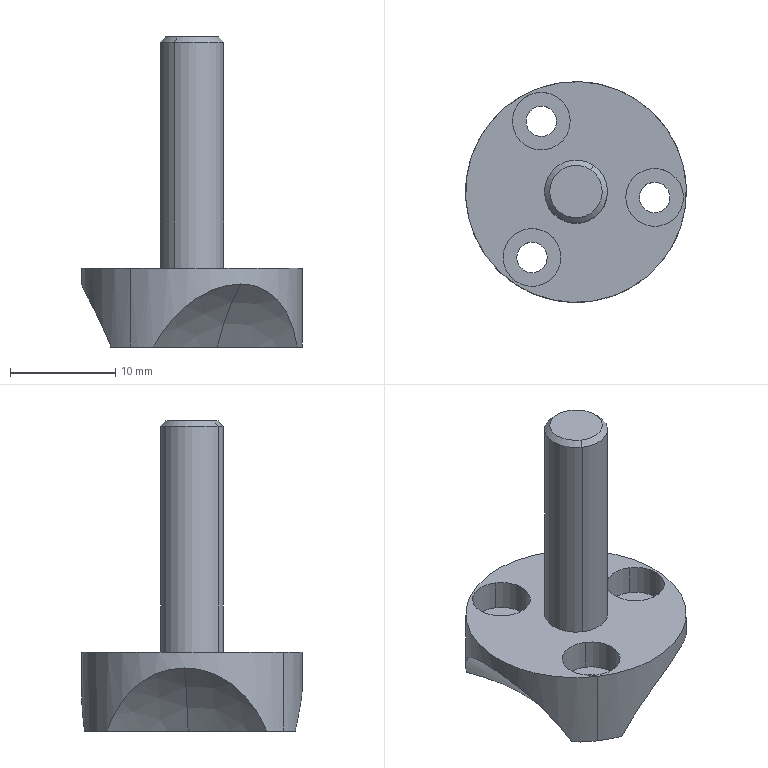Component | SolidWorks | Connector-1 | 1 solid | 33 faces | box 21 x 21 x 29.5 mm | volume 2358 mm3 | cylinder 18 | plane 7 | sphere 6 | cone 2 | commonest cylinder face diameters 5.5 x6 2.9 x6 10 x2 6 x2 21 x2
STEP:
#1=COLOUR_RGB('',0.7922,0.8196,0.9333);
#2=FILL_AREA_STYLE_COLOUR('',#1);
#3=FILL_AREA_STYLE('',(#2));
#4=SURFACE_STYLE_FILL_AREA(#3);
#5=SURFACE_SIDE_STYLE('',(#4));
#6=SURFACE_STYLE_USAGE(.BOTH.,#5);
#7=PRESENTATION_STYLE_ASSIGNMENT((#6));
#8=CARTESIAN_POINT('',(-8.497,3.918,42.455));
#9=VERTEX_POINT('',#8);
#10=CARTESIAN_POINT('',(-8.716,3.591,42.455));
#11=VERTEX_POINT('',#10);
#12=CARTESIAN_POINT('',(-8.607,3.755,42.455));
#13=DIRECTION('',(-0.,0.,-1.));
#14=DIRECTION('',(-0.5579,-0.8299,0.));
#15=AXIS2_PLACEMENT_3D('',#12,#13,#14);
#16=CIRCLE('',#15,0.1969);
#17=EDGE_CURVE('',#9,#11,#16,.T.);
#18=ORIENTED_EDGE('',*,*,#17,.F.);
#19=CARTESIAN_POINT('',(-8.497,3.918,42.396));
#20=VERTEX_POINT('',#19);
#21=CARTESIAN_POINT('',(-8.497,3.918,42.376));
#22=DIRECTION('',(-0.,0.,-1.));
#23=VECTOR('',#22,39.37);
#24=LINE('',#21,#23);
#25=EDGE_CURVE('',#9,#20,#24,.T.);
#26=ORIENTED_EDGE('',*,*,#25,.T.);
#27=CARTESIAN_POINT('',(-8.716,3.591,42.396));
#28=VERTEX_POINT('',#27);
#29=CARTESIAN_POINT('',(-8.607,3.755,42.396));
#30=DIRECTION('',(-0.,0.,-1.));
#31=DIRECTION('',(0.5579,0.8299,0.));
#32=AXIS2_PLACEMENT_3D('',#29,#30,#31);
#33=CIRCLE('',#32,0.1969);
#34=EDGE_CURVE('',#20,#28,#33,.T.);
#35=ORIENTED_EDGE('',*,*,#34,.T.);
#36=CARTESIAN_POINT('',(-8.716,3.591,42.376));
#37=DIRECTION('',(-0.,0.,-1.));
#38=VECTOR('',#37,39.37);
#39=LINE('',#36,#38);
#40=EDGE_CURVE('',#11,#28,#39,.T.);
#41=ORIENTED_EDGE('',*,*,#40,.F.);
#42=EDGE_LOOP('',(#18,#26,#35,#41));
#43=FACE_OUTER_BOUND('',#42,.T.);
#44=CARTESIAN_POINT('',(-8.607,3.755,42.376));
#45=DIRECTION('',(-0.,0.,-1.));
#46=DIRECTION('',(-0.5579,-0.8299,0.));
#47=AXIS2_PLACEMENT_3D('',#44,#45,#46);
#48=CYLINDRICAL_SURFACE('',#47,0.1969);
#49=ADVANCED_FACE('',(#43),#48,.F.);
#50=CARTESIAN_POINT('',(-8.821,3.769,42.396));
#51=VERTEX_POINT('',#50);
#52=CARTESIAN_POINT('',(-8.869,4.074,42.396));
#53=VERTEX_POINT('',#52);
#54=CARTESIAN_POINT('',(-9.51,3.816,42.396));
#55=DIRECTION('',(0.,-0.,1.));
#56=DIRECTION('',(0.5579,0.8299,0.));
#57=AXIS2_PLACEMENT_3D('',#54,#55,#56);
#58=CIRCLE('',#57,0.6906);
#59=EDGE_CURVE('',#51,#53,#58,.T.);
#60=ORIENTED_EDGE('',*,*,#59,.F.);
#61=CARTESIAN_POINT('',(-9.019,3.783,42.632));
#62=VERTEX_POINT('',#61);
#63=CARTESIAN_POINT('',(-9.51,3.816,42.017));
#64=DIRECTION('',(-0.06817,-0.9977,-0.));
#65=DIRECTION('',(0.9977,-0.06817,0.));
#66=AXIS2_PLACEMENT_3D('',#63,#64,#65);
#67=CIRCLE('',#66,0.7874);
#68=EDGE_CURVE('',#51,#62,#67,.T.);
#69=ORIENTED_EDGE('',*,*,#68,.T.);
#70=CARTESIAN_POINT('',(-9.019,3.783,42.632));
#71=CARTESIAN_POINT('',(-9.018,3.792,42.632));
#72=CARTESIAN_POINT('',(-9.017,3.801,42.631));
#73=CARTESIAN_POINT('',(-9.015,3.819,42.63));
#74=CARTESIAN_POINT('',(-9.014,3.827,42.628));
#75=CARTESIAN_POINT('',(-9.01,3.845,42.625));
#76=CARTESIAN_POINT('',(-9.008,3.853,42.623));
#77=CARTESIAN_POINT('',(-9.004,3.87,42.618));
#78=CARTESIAN_POINT('',(-9.001,3.878,42.615));
#79=CARTESIAN_POINT('',(-8.993,3.902,42.605));
#80=CARTESIAN_POINT('',(-8.987,3.917,42.598));
#81=CARTESIAN_POINT('',(-8.977,3.938,42.584));
#82=CARTESIAN_POINT('',(-8.974,3.945,42.579));
#83=CARTESIAN_POINT('',(-8.967,3.958,42.569));
#84=CARTESIAN_POINT('',(-8.963,3.964,42.564));
#85=CARTESIAN_POINT('',(-8.952,3.982,42.548));
#86=CARTESIAN_POINT('',(-8.944,3.993,42.536));
#87=CARTESIAN_POINT('',(-8.929,4.014,42.511));
#88=CARTESIAN_POINT('',(-8.921,4.023,42.498));
#89=CARTESIAN_POINT('',(-8.898,4.049,42.456));
#90=CARTESIAN_POINT('',(-8.883,4.062,42.427));
#91=CARTESIAN_POINT('',(-8.869,4.074,42.396));
#92=B_SPLINE_CURVE_WITH_KNOTS('',3,(#70,#71,#72,#73,#74,#75,#76,#77,#78,#79,#80,#81,#82,#83,#84,#85,#86,#87,#88,#89,#90,#91),.UNSPECIFIED.,.F.,.F.,(4,2,2,2,2,2,2,2,2,2,4),(0.01143,0.0121,0.01278,0.01346,0.01414,0.01549,0.01617,0.01684,0.0182,0.01955,0.02226),.UNSPECIFIED.);
#93=EDGE_CURVE('',#62,#53,#92,.T.);
#94=ORIENTED_EDGE('',*,*,#93,.T.);
#95=EDGE_LOOP('',(#60,#69,#94));
#96=FACE_OUTER_BOUND('',#95,.T.);
#97=CARTESIAN_POINT('',(-9.51,3.816,42.017));
#98=DIRECTION('',(0.06817,0.9977,0.));
#99=DIRECTION('',(0.9977,-0.06817,0.));
#100=AXIS2_PLACEMENT_3D('',#97,#98,#99);
#101=SPHERICAL_SURFACE('',#100,0.7874);
#102=ADVANCED_FACE('',(#96),#101,.F.);
#103=CARTESIAN_POINT('',(-8.512,3.561,42.396));
#104=VERTEX_POINT('',#103);
#105=CARTESIAN_POINT('',(-8.751,3.367,42.396));
#106=VERTEX_POINT('',#105);
#107=CARTESIAN_POINT('',(-8.208,2.941,42.396));
#108=DIRECTION('',(0.,-0.,1.));
#109=DIRECTION('',(0.5579,0.8299,0.));
#110=AXIS2_PLACEMENT_3D('',#107,#108,#109);
#111=CIRCLE('',#110,0.6906);
#112=EDGE_CURVE('',#104,#106,#111,.T.);
#113=ORIENTED_EDGE('',*,*,#112,.F.);
#114=CARTESIAN_POINT('',(-8.425,3.383,42.632));
#115=VERTEX_POINT('',#114);
#116=CARTESIAN_POINT('',(-8.208,2.941,42.017));
#117=DIRECTION('',(0.8981,0.4398,-0.));
#118=DIRECTION('',(-0.4398,0.8981,0.));
#119=AXIS2_PLACEMENT_3D('',#116,#117,#118);
#120=CIRCLE('',#119,0.7874);
#121=EDGE_CURVE('',#104,#115,#120,.T.);
#122=ORIENTED_EDGE('',*,*,#121,.T.);
#123=CARTESIAN_POINT('',(-8.425,3.383,42.632));
#124=CARTESIAN_POINT('',(-8.433,3.379,42.632));
#125=CARTESIAN_POINT('',(-8.441,3.376,42.631));
#126=CARTESIAN_POINT('',(-8.458,3.369,42.63));
#127=CARTESIAN_POINT('',(-8.466,3.366,42.628));
#128=CARTESIAN_POINT('',(-8.483,3.36,42.625));
#129=CARTESIAN_POINT('',(-8.491,3.358,42.623));
#130=CARTESIAN_POINT('',(-8.508,3.353,42.618));
#131=CARTESIAN_POINT('',(-8.516,3.351,42.615));
#132=CARTESIAN_POINT('',(-8.541,3.346,42.605));
#133=CARTESIAN_POINT('',(-8.557,3.344,42.598));
#134=CARTESIAN_POINT('',(-8.58,3.342,42.584));
#135=CARTESIAN_POINT('',(-8.588,3.342,42.579));
#136=CARTESIAN_POINT('',(-8.603,3.341,42.569));
#137=CARTESIAN_POINT('',(-8.61,3.341,42.564));
#138=CARTESIAN_POINT('',(-8.631,3.342,42.548));
#139=CARTESIAN_POINT('',(-8.644,3.343,42.536));
#140=CARTESIAN_POINT('',(-8.67,3.346,42.511));
#141=CARTESIAN_POINT('',(-8.682,3.348,42.498));
#142=CARTESIAN_POINT('',(-8.715,3.355,42.456));
#143=CARTESIAN_POINT('',(-8.735,3.361,42.427));
#144=CARTESIAN_POINT('',(-8.751,3.367,42.396));
#145=B_SPLINE_CURVE_WITH_KNOTS('',3,(#123,#124,#125,#126,#127,#128,#129,#130,#131,#132,#133,#134,#135,#136,#137,#138,#139,#140,#141,#142,#143,#144),.UNSPECIFIED.,.F.,.F.,(4,2,2,2,2,2,2,2,2,2,4),(0.01143,0.0121,0.01278,0.01346,0.01414,0.01549,0.01617,0.01684,0.0182,0.01955,0.02226),.UNSPECIFIED.);
#146=EDGE_CURVE('',#115,#106,#145,.T.);
#147=ORIENTED_EDGE('',*,*,#146,.T.);
#148=EDGE_LOOP('',(#113,#122,#147));
#149=FACE_OUTER_BOUND('',#148,.T.);
#150=CARTESIAN_POINT('',(-8.208,2.941,42.017));
#151=DIRECTION('',(-0.8981,-0.4398,0.));
#152=DIRECTION('',(-0.4398,0.8981,0.));
#153=AXIS2_PLACEMENT_3D('',#150,#151,#152);
#154=SPHERICAL_SURFACE('',#153,0.7874);
#155=ADVANCED_FACE('',(#149),#154,.F.);
#156=CARTESIAN_POINT('',(-8.487,3.933,42.396));
#157=VERTEX_POINT('',#156);
#158=CARTESIAN_POINT('',(-8.199,3.823,42.396));
#159=VERTEX_POINT('',#158);
#160=CARTESIAN_POINT('',(-8.101,4.506,42.396));
#161=DIRECTION('',(0.,-0.,1.));
#162=DIRECTION('',(0.5579,0.8299,0.));
#163=AXIS2_PLACEMENT_3D('',#160,#161,#162);
#164=CIRCLE('',#163,0.6906);
#165=EDGE_CURVE('',#157,#159,#164,.T.);
#166=ORIENTED_EDGE('',*,*,#165,.F.);
#167=CARTESIAN_POINT('',(-8.376,4.098,42.632));
#168=VERTEX_POINT('',#167);
#169=CARTESIAN_POINT('',(-8.101,4.506,42.017));
#170=DIRECTION('',(-0.8299,0.5579,0.));
#171=DIRECTION('',(-0.5579,-0.8299,0.));
#172=AXIS2_PLACEMENT_3D('',#169,#170,#171);
#173=CIRCLE('',#172,0.7874);
#174=EDGE_CURVE('',#157,#168,#173,.T.);
#175=ORIENTED_EDGE('',*,*,#174,.T.);
#176=CARTESIAN_POINT('',(-8.376,4.098,42.632));
#177=CARTESIAN_POINT('',(-8.368,4.093,42.632));
#178=CARTESIAN_POINT('',(-8.361,4.087,42.631));
#179=CARTESIAN_POINT('',(-8.347,4.076,42.63));
#180=CARTESIAN_POINT('',(-8.34,4.071,42.628));
#181=CARTESIAN_POINT('',(-8.327,4.059,42.625));
#182=CARTESIAN_POINT('',(-8.321,4.053,42.623));
#183=CARTESIAN_POINT('',(-8.308,4.041,42.618));
#184=CARTESIAN_POINT('',(-8.302,4.035,42.615));
#185=CARTESIAN_POINT('',(-8.286,4.016,42.605));
#186=CARTESIAN_POINT('',(-8.276,4.003,42.598));
#187=CARTESIAN_POINT('',(-8.262,3.984,42.584));
#188=CARTESIAN_POINT('',(-8.258,3.977,42.579));
#189=CARTESIAN_POINT('',(-8.25,3.965,42.569));
#190=CARTESIAN_POINT('',(-8.247,3.958,42.564));
#191=CARTESIAN_POINT('',(-8.237,3.94,42.548));
#192=CARTESIAN_POINT('',(-8.231,3.928,42.536));
#193=CARTESIAN_POINT('',(-8.221,3.904,42.511));
#194=CARTESIAN_POINT('',(-8.217,3.893,42.498));
#195=CARTESIAN_POINT('',(-8.206,3.86,42.456));
#196=CARTESIAN_POINT('',(-8.202,3.84,42.427));
#197=CARTESIAN_POINT('',(-8.199,3.823,42.396));
#198=B_SPLINE_CURVE_WITH_KNOTS('',3,(#176,#177,#178,#179,#180,#181,#182,#183,#184,#185,#186,#187,#188,#189,#190,#191,#192,#193,#194,#195,#196,#197),.UNSPECIFIED.,.F.,.F.,(4,2,2,2,2,2,2,2,2,2,4),(0.01143,0.0121,0.01278,0.01346,0.01414,0.01549,0.01617,0.01684,0.0182,0.01955,0.02226),.UNSPECIFIED.);
#199=EDGE_CURVE('',#168,#159,#198,.T.);
#200=ORIENTED_EDGE('',*,*,#199,.T.);
#201=EDGE_LOOP('',(#166,#175,#200));
#202=FACE_OUTER_BOUND('',#201,.T.);
#203=CARTESIAN_POINT('',(-8.101,4.506,42.017));
#204=DIRECTION('',(0.8299,-0.5579,-0.));
#205=DIRECTION('',(-0.5579,-0.8299,0.));
#206=AXIS2_PLACEMENT_3D('',#203,#204,#205);
#207=SPHERICAL_SURFACE('',#206,0.7874);
#208=ADVANCED_FACE('',(#202),#207,.F.);
#209=CARTESIAN_POINT('',(-8.832,3.42,42.577));
#210=VERTEX_POINT('',#209);
#211=CARTESIAN_POINT('',(-8.711,3.599,42.577));
#212=VERTEX_POINT('',#211);
#213=CARTESIAN_POINT('',(-8.771,3.51,42.577));
#214=DIRECTION('',(0.,-0.,1.));
#215=DIRECTION('',(0.5579,0.8299,0.));
#216=AXIS2_PLACEMENT_3D('',#213,#214,#215);
#217=CIRCLE('',#216,0.1083);
#218=EDGE_CURVE('',#210,#212,#217,.T.);
#219=ORIENTED_EDGE('',*,*,#218,.F.);
#220=CARTESIAN_POINT('',(-8.832,3.42,42.691));
#221=VERTEX_POINT('',#220);
#222=CARTESIAN_POINT('',(-8.832,3.42,42.691));
#223=DIRECTION('',(0.,-0.,1.));
#224=VECTOR('',#223,39.37);
#225=LINE('',#222,#224);
#226=EDGE_CURVE('',#210,#221,#225,.T.);
#227=ORIENTED_EDGE('',*,*,#226,.T.);
#228=CARTESIAN_POINT('',(-8.711,3.599,42.691));
#229=VERTEX_POINT('',#228);
#230=CARTESIAN_POINT('',(-8.771,3.51,42.691));
#231=DIRECTION('',(0.,-0.,1.));
#232=DIRECTION('',(0.5579,0.8299,0.));
#233=AXIS2_PLACEMENT_3D('',#230,#231,#232);
#234=CIRCLE('',#233,0.1083);
#235=EDGE_CURVE('',#221,#229,#234,.T.);
#236=ORIENTED_EDGE('',*,*,#235,.T.);
#237=CARTESIAN_POINT('',(-8.711,3.599,42.691));
#238=DIRECTION('',(0.,-0.,1.));
#239=VECTOR('',#238,39.37);
#240=LINE('',#237,#239);
#241=EDGE_CURVE('',#212,#229,#240,.T.);
#242=ORIENTED_EDGE('',*,*,#241,.F.);
#243=EDGE_LOOP('',(#219,#227,#236,#242));
#244=FACE_OUTER_BOUND('',#243,.T.);
#245=CARTESIAN_POINT('',(-8.771,3.51,42.691));
#246=DIRECTION('',(0.,-0.,1.));
#247=DIRECTION('',(0.5579,0.8299,0.));
#248=AXIS2_PLACEMENT_3D('',#245,#246,#247);
#249=CYLINDRICAL_SURFACE('',#248,0.1083);
#250=ADVANCED_FACE('',(#244),#249,.F.);
#251=CARTESIAN_POINT('',(-8.739,3.557,42.396));
#252=VERTEX_POINT('',#251);
#253=CARTESIAN_POINT('',(-8.803,3.462,42.396));
#254=VERTEX_POINT('',#253);
#255=CARTESIAN_POINT('',(-8.771,3.51,42.396));
#256=DIRECTION('',(-0.,0.,-1.));
#257=DIRECTION('',(0.5579,0.8299,0.));
#258=AXIS2_PLACEMENT_3D('',#255,#256,#257);
#259=CIRCLE('',#258,0.05709);
#260=EDGE_CURVE('',#252,#254,#259,.T.);
#261=ORIENTED_EDGE('',*,*,#260,.T.);
#262=CARTESIAN_POINT('',(-8.803,3.462,42.577));
#263=VERTEX_POINT('',#262);
#264=CARTESIAN_POINT('',(-8.803,3.462,42.691));
#265=DIRECTION('',(0.,-0.,1.));
#266=VECTOR('',#265,39.37);
#267=LINE('',#264,#266);
#268=EDGE_CURVE('',#254,#263,#267,.T.);
#269=ORIENTED_EDGE('',*,*,#268,.T.);
#270=CARTESIAN_POINT('',(-8.739,3.557,42.577));
#271=VERTEX_POINT('',#270);
#272=CARTESIAN_POINT('',(-8.771,3.51,42.577));
#273=DIRECTION('',(0.,-0.,1.));
#274=DIRECTION('',(0.5579,0.8299,0.));
#275=AXIS2_PLACEMENT_3D('',#272,#273,#274);
#276=CIRCLE('',#275,0.05709);
#277=EDGE_CURVE('',#263,#271,#276,.T.);
#278=ORIENTED_EDGE('',*,*,#277,.T.);
#279=CARTESIAN_POINT('',(-8.739,3.557,42.691));
#280=DIRECTION('',(0.,-0.,1.));
#281=VECTOR('',#280,39.37);
#282=LINE('',#279,#281);
#283=EDGE_CURVE('',#252,#271,#282,.T.);
#284=ORIENTED_EDGE('',*,*,#283,.F.);
#285=EDGE_LOOP('',(#261,#269,#278,#284));
#286=FACE_OUTER_BOUND('',#285,.T.);
#287=CARTESIAN_POINT('',(-8.771,3.51,42.691));
#288=DIRECTION('',(0.,-0.,1.));
#289=DIRECTION('',(0.5579,0.8299,0.));
#290=AXIS2_PLACEMENT_3D('',#287,#288,#289);
#291=CYLINDRICAL_SURFACE('',#290,0.05709);
#292=ADVANCED_FACE('',(#286),#291,.F.);
#293=CARTESIAN_POINT('',(-8.797,3.93,42.577));
#294=VERTEX_POINT('',#293);
#295=CARTESIAN_POINT('',(-8.676,4.11,42.577));
#296=VERTEX_POINT('',#295);
#297=CARTESIAN_POINT('',(-8.736,4.02,42.577));
#298=DIRECTION('',(0.,-0.,1.));
#299=DIRECTION('',(0.5579,0.8299,0.));
#300=AXIS2_PLACEMENT_3D('',#297,#298,#299);
#301=CIRCLE('',#300,0.1083);
#302=EDGE_CURVE('',#294,#296,#301,.T.);
#303=ORIENTED_EDGE('',*,*,#302,.F.);
#304=CARTESIAN_POINT('',(-8.797,3.93,42.691));
#305=VERTEX_POINT('',#304);
#306=CARTESIAN_POINT('',(-8.797,3.93,42.691));
#307=DIRECTION('',(0.,-0.,1.));
#308=VECTOR('',#307,39.37);
#309=LINE('',#306,#308);
#310=EDGE_CURVE('',#294,#305,#309,.T.);
#311=ORIENTED_EDGE('',*,*,#310,.T.);
#312=CARTESIAN_POINT('',(-8.676,4.11,42.691));
#313=VERTEX_POINT('',#312);
#314=CARTESIAN_POINT('',(-8.736,4.02,42.691));
#315=DIRECTION('',(0.,-0.,1.));
#316=DIRECTION('',(0.5579,0.8299,0.));
#317=AXIS2_PLACEMENT_3D('',#314,#315,#316);
#318=CIRCLE('',#317,0.1083);
#319=EDGE_CURVE('',#305,#313,#318,.T.);
#320=ORIENTED_EDGE('',*,*,#319,.T.);
#321=CARTESIAN_POINT('',(-8.676,4.11,42.691));
#322=DIRECTION('',(0.,-0.,1.));
#323=VECTOR('',#322,39.37);
#324=LINE('',#321,#323);
#325=EDGE_CURVE('',#296,#313,#324,.T.);
#326=ORIENTED_EDGE('',*,*,#325,.F.);
#327=EDGE_LOOP('',(#303,#311,#320,#326));
#328=FACE_OUTER_BOUND('',#327,.T.);
#329=CARTESIAN_POINT('',(-8.736,4.02,42.691));
#330=DIRECTION('',(0.,-0.,1.));
#331=DIRECTION('',(0.5579,0.8299,0.));
#332=AXIS2_PLACEMENT_3D('',#329,#330,#331);
#333=CYLINDRICAL_SURFACE('',#332,0.1083);
#334=ADVANCED_FACE('',(#328),#333,.F.);
#335=CARTESIAN_POINT('',(-8.705,4.067,42.396));
#336=VERTEX_POINT('',#335);
#337=CARTESIAN_POINT('',(-8.768,3.972,42.396));
#338=VERTEX_POINT('',#337);
#339=CARTESIAN_POINT('',(-8.736,4.02,42.396));
#340=DIRECTION('',(-0.,0.,-1.));
#341=DIRECTION('',(0.5579,0.8299,0.));
#342=AXIS2_PLACEMENT_3D('',#339,#340,#341);
#343=CIRCLE('',#342,0.05709);
#344=EDGE_CURVE('',#336,#338,#343,.T.);
#345=ORIENTED_EDGE('',*,*,#344,.T.);
#346=CARTESIAN_POINT('',(-8.768,3.972,42.577));
#347=VERTEX_POINT('',#346);
#348=CARTESIAN_POINT('',(-8.768,3.972,42.691));
#349=DIRECTION('',(0.,-0.,1.));
#350=VECTOR('',#349,39.37);
#351=LINE('',#348,#350);
#352=EDGE_CURVE('',#338,#347,#351,.T.);
#353=ORIENTED_EDGE('',*,*,#352,.T.);
#354=CARTESIAN_POINT('',(-8.705,4.067,42.577));
#355=VERTEX_POINT('',#354);
#356=CARTESIAN_POINT('',(-8.736,4.02,42.577));
#357=DIRECTION('',(0.,-0.,1.));
#358=DIRECTION('',(0.5579,0.8299,0.));
#359=AXIS2_PLACEMENT_3D('',#356,#357,#358);
#360=CIRCLE('',#359,0.05709);
#361=EDGE_CURVE('',#347,#355,#360,.T.);
#362=ORIENTED_EDGE('',*,*,#361,.T.);
#363=CARTESIAN_POINT('',(-8.705,4.067,42.691));
#364=DIRECTION('',(0.,-0.,1.));
#365=VECTOR('',#364,39.37);
#366=LINE('',#363,#365);
#367=EDGE_CURVE('',#336,#355,#366,.T.);
#368=ORIENTED_EDGE('',*,*,#367,.F.);
#369=EDGE_LOOP('',(#345,#353,#362,#368));
#370=FACE_OUTER_BOUND('',#369,.T.);
#371=CARTESIAN_POINT('',(-8.736,4.02,42.691));
#372=DIRECTION('',(0.,-0.,1.));
#373=DIRECTION('',(0.5579,0.8299,0.));
#374=AXIS2_PLACEMENT_3D('',#371,#372,#373);
#375=CYLINDRICAL_SURFACE('',#374,0.05709);
#376=ADVANCED_FACE('',(#370),#375,.F.);
#377=CARTESIAN_POINT('',(-8.372,3.645,42.577));
#378=VERTEX_POINT('',#377);
#379=CARTESIAN_POINT('',(-8.252,3.824,42.577));
#380=VERTEX_POINT('',#379);
#381=CARTESIAN_POINT('',(-8.312,3.734,42.577));
#382=DIRECTION('',(0.,-0.,1.));
#383=DIRECTION('',(0.5579,0.8299,0.));
#384=AXIS2_PLACEMENT_3D('',#381,#382,#383);
#385=CIRCLE('',#384,0.1083);
#386=EDGE_CURVE('',#378,#380,#385,.T.);
#387=ORIENTED_EDGE('',*,*,#386,.F.);
#388=CARTESIAN_POINT('',(-8.372,3.645,42.691));
#389=VERTEX_POINT('',#388);
#390=CARTESIAN_POINT('',(-8.372,3.645,42.691));
#391=DIRECTION('',(0.,-0.,1.));
#392=VECTOR('',#391,39.37);
#393=LINE('',#390,#392);
#394=EDGE_CURVE('',#378,#389,#393,.T.);
#395=ORIENTED_EDGE('',*,*,#394,.T.);
#396=CARTESIAN_POINT('',(-8.252,3.824,42.691));
#397=VERTEX_POINT('',#396);
#398=CARTESIAN_POINT('',(-8.312,3.734,42.691));
#399=DIRECTION('',(0.,-0.,1.));
#400=DIRECTION('',(0.5579,0.8299,0.));
#401=AXIS2_PLACEMENT_3D('',#398,#399,#400);
#402=CIRCLE('',#401,0.1083);
#403=EDGE_CURVE('',#389,#397,#402,.T.);
#404=ORIENTED_EDGE('',*,*,#403,.T.);
#405=CARTESIAN_POINT('',(-8.252,3.824,42.691));
#406=DIRECTION('',(0.,-0.,1.));
#407=VECTOR('',#406,39.37);
#408=LINE('',#405,#407);
#409=EDGE_CURVE('',#380,#397,#408,.T.);
#410=ORIENTED_EDGE('',*,*,#409,.F.);
#411=EDGE_LOOP('',(#387,#395,#404,#410));
#412=FACE_OUTER_BOUND('',#411,.T.);
#413=CARTESIAN_POINT('',(-8.312,3.734,42.691));
#414=DIRECTION('',(0.,-0.,1.));
#415=DIRECTION('',(0.5579,0.8299,0.));
#416=AXIS2_PLACEMENT_3D('',#413,#414,#415);
#417=CYLINDRICAL_SURFACE('',#416,0.1083);
#418=ADVANCED_FACE('',(#412),#417,.F.);
#419=CARTESIAN_POINT('',(-8.28,3.782,42.396));
#420=VERTEX_POINT('',#419);
#421=CARTESIAN_POINT('',(-8.344,3.687,42.396));
#422=VERTEX_POINT('',#421);
#423=CARTESIAN_POINT('',(-8.312,3.734,42.396));
#424=DIRECTION('',(-0.,0.,-1.));
#425=DIRECTION('',(0.5579,0.8299,0.));
#426=AXIS2_PLACEMENT_3D('',#423,#424,#425);
#427=CIRCLE('',#426,0.05709);
#428=EDGE_CURVE('',#420,#422,#427,.T.);
#429=ORIENTED_EDGE('',*,*,#428,.T.);
#430=CARTESIAN_POINT('',(-8.344,3.687,42.577));
#431=VERTEX_POINT('',#430);
#432=CARTESIAN_POINT('',(-8.344,3.687,42.691));
#433=DIRECTION('',(0.,-0.,1.));
#434=VECTOR('',#433,39.37);
#435=LINE('',#432,#434);
#436=EDGE_CURVE('',#422,#431,#435,.T.);
#437=ORIENTED_EDGE('',*,*,#436,.T.);
#438=CARTESIAN_POINT('',(-8.28,3.782,42.577));
#439=VERTEX_POINT('',#438);
#440=CARTESIAN_POINT('',(-8.312,3.734,42.577));
#441=DIRECTION('',(0.,-0.,1.));
#442=DIRECTION('',(0.5579,0.8299,0.));
#443=AXIS2_PLACEMENT_3D('',#440,#441,#442);
#444=CIRCLE('',#443,0.05709);
#445=EDGE_CURVE('',#431,#439,#444,.T.);
#446=ORIENTED_EDGE('',*,*,#445,.T.);
#447=CARTESIAN_POINT('',(-8.28,3.782,42.691));
#448=DIRECTION('',(0.,-0.,1.));
#449=VECTOR('',#448,39.37);
#450=LINE('',#447,#449);
#451=EDGE_CURVE('',#420,#439,#450,.T.);
#452=ORIENTED_EDGE('',*,*,#451,.F.);
#453=EDGE_LOOP('',(#429,#437,#446,#452));
#454=FACE_OUTER_BOUND('',#453,.T.);
#455=CARTESIAN_POINT('',(-8.312,3.734,42.691));
#456=DIRECTION('',(0.,-0.,1.));
#457=DIRECTION('',(0.5579,0.8299,0.));
#458=AXIS2_PLACEMENT_3D('',#455,#456,#457);
#459=CYLINDRICAL_SURFACE('',#458,0.05709);
#460=ADVANCED_FACE('',(#454),#459,.F.);
#461=CARTESIAN_POINT('',(-8.552,3.836,43.557));
#462=VERTEX_POINT('',#461);
#463=CARTESIAN_POINT('',(-8.661,3.673,43.557));
#464=VERTEX_POINT('',#463);
#465=CARTESIAN_POINT('',(-8.607,3.755,43.557));
#466=DIRECTION('',(0.,-0.,1.));
#467=DIRECTION('',(-0.5579,-0.8299,0.));
#468=AXIS2_PLACEMENT_3D('',#465,#466,#467);
#469=CIRCLE('',#468,0.09843);
#470=EDGE_CURVE('',#462,#464,#469,.T.);
#471=ORIENTED_EDGE('',*,*,#470,.F.);
#472=CARTESIAN_POINT('',(-8.541,3.853,43.537));
#473=VERTEX_POINT('',#472);
#474=CARTESIAN_POINT('',(-8.541,3.853,43.537));
#475=DIRECTION('',(0.3945,0.5868,-0.7071));
#476=VECTOR('',#475,39.37);
#477=LINE('',#474,#476);
#478=EDGE_CURVE('',#462,#473,#477,.T.);
#479=ORIENTED_EDGE('',*,*,#478,.T.);
#480=CARTESIAN_POINT('',(-8.672,3.657,43.537));
#481=VERTEX_POINT('',#480);
#482=CARTESIAN_POINT('',(-8.607,3.755,43.537));
#483=DIRECTION('',(-0.,0.,-1.));
#484=DIRECTION('',(-0.5579,-0.8299,0.));
#485=AXIS2_PLACEMENT_3D('',#482,#483,#484);
#486=CIRCLE('',#485,0.1181);
#487=EDGE_CURVE('',#481,#473,#486,.T.);
#488=ORIENTED_EDGE('',*,*,#487,.F.);
#489=CARTESIAN_POINT('',(-8.672,3.657,43.537));
#490=DIRECTION('',(-0.3945,-0.5868,-0.7071));
#491=VECTOR('',#490,39.37);
#492=LINE('',#489,#491);
#493=EDGE_CURVE('',#464,#481,#492,.T.);
#494=ORIENTED_EDGE('',*,*,#493,.F.);
#495=EDGE_LOOP('',(#471,#479,#488,#494));
#496=FACE_OUTER_BOUND('',#495,.T.);
#497=CARTESIAN_POINT('',(-8.607,3.755,43.537));
#498=DIRECTION('',(-0.,0.,-1.));
#499=DIRECTION('',(-0.5579,-0.8299,0.));
#500=AXIS2_PLACEMENT_3D('',#497,#498,#499);
#501=CONICAL_SURFACE('',#500,0.1181,0.7854);
#502=ADVANCED_FACE('',(#496),#501,.T.);
#503=ORIENTED_EDGE('',*,*,#487,.T.);
#504=CARTESIAN_POINT('',(-8.541,3.853,42.691));
#505=VERTEX_POINT('',#504);
#506=CARTESIAN_POINT('',(-8.541,3.853,42.376));
#507=DIRECTION('',(-0.,0.,-1.));
#508=VECTOR('',#507,39.37);
#509=LINE('',#506,#508);
#510=EDGE_CURVE('',#473,#505,#509,.T.);
#511=ORIENTED_EDGE('',*,*,#510,.T.);
#512=CARTESIAN_POINT('',(-8.672,3.657,42.691));
#513=VERTEX_POINT('',#512);
#514=CARTESIAN_POINT('',(-8.607,3.755,42.691));
#515=DIRECTION('',(-0.,0.,-1.));
#516=DIRECTION('',(-0.5579,-0.8299,0.));
#517=AXIS2_PLACEMENT_3D('',#514,#515,#516);
#518=CIRCLE('',#517,0.1181);
#519=EDGE_CURVE('',#513,#505,#518,.T.);
#520=ORIENTED_EDGE('',*,*,#519,.F.);
#521=CARTESIAN_POINT('',(-8.672,3.657,42.376));
#522=DIRECTION('',(-0.,0.,-1.));
#523=VECTOR('',#522,39.37);
#524=LINE('',#521,#523);
#525=EDGE_CURVE('',#481,#513,#524,.T.);
#526=ORIENTED_EDGE('',*,*,#525,.F.);
#527=EDGE_LOOP('',(#503,#511,#520,#526));
#528=FACE_OUTER_BOUND('',#527,.T.);
#529=CARTESIAN_POINT('',(-8.607,3.755,42.376));
#530=DIRECTION('',(-0.,0.,-1.));
#531=DIRECTION('',(-0.5579,-0.8299,0.));
#532=AXIS2_PLACEMENT_3D('',#529,#530,#531);
#533=CYLINDRICAL_SURFACE('',#532,0.1181);
#534=ADVANCED_FACE('',(#528),#533,.T.);
#535=CARTESIAN_POINT('',(-8.837,3.412,42.691));
#536=VERTEX_POINT('',#535);
#537=CARTESIAN_POINT('',(-8.376,4.098,42.691));
#538=VERTEX_POINT('',#537);
#539=CARTESIAN_POINT('',(-8.607,3.755,42.691));
#540=DIRECTION('',(-0.,0.,-1.));
#541=DIRECTION('',(-0.5579,-0.8299,0.));
#542=AXIS2_PLACEMENT_3D('',#539,#540,#541);
#543=CIRCLE('',#542,0.4134);
#544=EDGE_CURVE('',#536,#538,#543,.T.);
#545=ORIENTED_EDGE('',*,*,#544,.T.);
#546=CARTESIAN_POINT('',(-8.376,4.098,42.376));
#547=DIRECTION('',(-0.,0.,-1.));
#548=VECTOR('',#547,39.37);
#549=LINE('',#546,#548);
#550=EDGE_CURVE('',#538,#168,#549,.T.);
#551=ORIENTED_EDGE('',*,*,#550,.T.);
#552=CARTESIAN_POINT('',(-8.697,4.158,42.396));
#553=VERTEX_POINT('',#552);
#554=CARTESIAN_POINT('',(-8.697,4.158,42.396));
#555=CARTESIAN_POINT('',(-8.68,4.162,42.427));
#556=CARTESIAN_POINT('',(-8.66,4.165,42.456));
#557=CARTESIAN_POINT('',(-8.626,4.168,42.497));
#558=CARTESIAN_POINT('',(-8.614,4.168,42.511));
#559=CARTESIAN_POINT('',(-8.588,4.168,42.536));
#560=CARTESIAN_POINT('',(-8.575,4.167,42.548));
#561=CARTESIAN_POINT('',(-8.546,4.164,42.57));
#562=CARTESIAN_POINT('',(-8.532,4.161,42.58));
#563=CARTESIAN_POINT('',(-8.501,4.155,42.598));
#564=CARTESIAN_POINT('',(-8.486,4.15,42.606));
#565=CARTESIAN_POINT('',(-8.454,4.139,42.618));
#566=CARTESIAN_POINT('',(-8.438,4.132,42.623));
#567=CARTESIAN_POINT('',(-8.406,4.117,42.63));
#568=CARTESIAN_POINT('',(-8.391,4.108,42.632));
#569=CARTESIAN_POINT('',(-8.376,4.098,42.632));
#570=B_SPLINE_CURVE_WITH_KNOTS('',3,(#554,#555,#556,#557,#558,#559,#560,#561,#562,#563,#564,#565,#566,#567,#568,#569),.UNSPECIFIED.,.F.,.F.,(4,2,2,2,2,2,2,4),(0.0005666,0.003282,0.004639,0.005997,0.007355,0.008712,0.01007,0.01143),.UNSPECIFIED.);
#571=EDGE_CURVE('',#553,#168,#570,.T.);
#572=ORIENTED_EDGE('',*,*,#571,.F.);
#573=CARTESIAN_POINT('',(-8.607,3.755,42.396));
#574=DIRECTION('',(0.,-0.,1.));
#575=DIRECTION('',(0.5579,0.8299,0.));
#576=AXIS2_PLACEMENT_3D('',#573,#574,#575);
#577=CIRCLE('',#576,0.4134);
#578=EDGE_CURVE('',#553,#53,#577,.T.);
#579=ORIENTED_EDGE('',*,*,#578,.T.);
#580=ORIENTED_EDGE('',*,*,#93,.F.);
#581=CARTESIAN_POINT('',(-8.91,3.474,42.396));
#582=VERTEX_POINT('',#581);
#583=CARTESIAN_POINT('',(-8.91,3.474,42.396));
#584=CARTESIAN_POINT('',(-8.922,3.487,42.427));
#585=CARTESIAN_POINT('',(-8.935,3.503,42.456));
#586=CARTESIAN_POINT('',(-8.955,3.531,42.497));
#587=CARTESIAN_POINT('',(-8.961,3.542,42.511));
#588=CARTESIAN_POINT('',(-8.974,3.564,42.536));
#589=CARTESIAN_POINT('',(-8.98,3.576,42.548));
#590=CARTESIAN_POINT('',(-8.991,3.602,42.57));
#591=CARTESIAN_POINT('',(-8.996,3.616,42.58));
#592=CARTESIAN_POINT('',(-9.006,3.646,42.598));
#593=CARTESIAN_POINT('',(-9.01,3.662,42.606));
#594=CARTESIAN_POINT('',(-9.016,3.694,42.618));
#595=CARTESIAN_POINT('',(-9.018,3.712,42.623));
#596=CARTESIAN_POINT('',(-9.02,3.747,42.63));
#597=CARTESIAN_POINT('',(-9.02,3.765,42.632));
#598=CARTESIAN_POINT('',(-9.019,3.783,42.632));
#599=B_SPLINE_CURVE_WITH_KNOTS('',3,(#583,#584,#585,#586,#587,#588,#589,#590,#591,#592,#593,#594,#595,#596,#597,#598),.UNSPECIFIED.,.F.,.F.,(4,2,2,2,2,2,2,4),(0.0005666,0.003282,0.004639,0.005997,0.007355,0.008712,0.01007,0.01143),.UNSPECIFIED.);
#600=EDGE_CURVE('',#582,#62,#599,.T.);
#601=ORIENTED_EDGE('',*,*,#600,.F.);
#602=CARTESIAN_POINT('',(-8.837,3.412,42.396));
#603=VERTEX_POINT('',#602);
#604=CARTESIAN_POINT('',(-8.607,3.755,42.396));
#605=DIRECTION('',(0.,-0.,1.));
#606=DIRECTION('',(0.5579,0.8299,0.));
#607=AXIS2_PLACEMENT_3D('',#604,#605,#606);
#608=CIRCLE('',#607,0.4134);
#609=EDGE_CURVE('',#582,#603,#608,.T.);
#610=ORIENTED_EDGE('',*,*,#609,.T.);
#611=CARTESIAN_POINT('',(-8.837,3.412,42.376));
#612=DIRECTION('',(-0.,0.,-1.));
#613=VECTOR('',#612,39.37);
#614=LINE('',#611,#613);
#615=EDGE_CURVE('',#536,#603,#614,.T.);
#616=ORIENTED_EDGE('',*,*,#615,.F.);
#617=EDGE_LOOP('',(#545,#551,#572,#579,#580,#601,#610,#616));
#618=FACE_OUTER_BOUND('',#617,.T.);
#619=CARTESIAN_POINT('',(-8.607,3.755,42.376));
#620=DIRECTION('',(-0.,0.,-1.));
#621=DIRECTION('',(-0.5579,-0.8299,0.));
#622=AXIS2_PLACEMENT_3D('',#619,#620,#621);
#623=CYLINDRICAL_SURFACE('',#622,0.4134);
#624=ADVANCED_FACE('',(#618),#623,.T.);
#625=ORIENTED_EDGE('',*,*,#550,.F.);
#626=CARTESIAN_POINT('',(-8.607,3.755,42.691));
#627=DIRECTION('',(-0.,0.,-1.));
#628=DIRECTION('',(-0.5579,-0.8299,0.));
#629=AXIS2_PLACEMENT_3D('',#626,#627,#628);
#630=CIRCLE('',#629,0.4134);
#631=EDGE_CURVE('',#538,#536,#630,.T.);
#632=ORIENTED_EDGE('',*,*,#631,.T.);
#633=ORIENTED_EDGE('',*,*,#615,.T.);
#634=CARTESIAN_POINT('',(-8.607,3.755,42.396));
#635=DIRECTION('',(0.,-0.,1.));
#636=DIRECTION('',(0.5579,0.8299,0.));
#637=AXIS2_PLACEMENT_3D('',#634,#635,#636);
#638=CIRCLE('',#637,0.4134);
#639=EDGE_CURVE('',#603,#106,#638,.T.);
#640=ORIENTED_EDGE('',*,*,#639,.T.);
#641=ORIENTED_EDGE('',*,*,#146,.F.);
#642=CARTESIAN_POINT('',(-8.212,3.632,42.396));
#643=VERTEX_POINT('',#642);
#644=CARTESIAN_POINT('',(-8.212,3.632,42.396));
#645=CARTESIAN_POINT('',(-8.217,3.615,42.427));
#646=CARTESIAN_POINT('',(-8.224,3.596,42.456));
#647=CARTESIAN_POINT('',(-8.239,3.565,42.497));
#648=CARTESIAN_POINT('',(-8.245,3.554,42.511));
#649=CARTESIAN_POINT('',(-8.258,3.532,42.536));
#650=CARTESIAN_POINT('',(-8.265,3.521,42.548));
#651=CARTESIAN_POINT('',(-8.282,3.498,42.57));
#652=CARTESIAN_POINT('',(-8.292,3.486,42.58));
#653=CARTESIAN_POINT('',(-8.313,3.463,42.598));
#654=CARTESIAN_POINT('',(-8.324,3.452,42.606));
#655=CARTESIAN_POINT('',(-8.35,3.43,42.618));
#656=CARTESIAN_POINT('',(-8.364,3.42,42.623));
#657=CARTESIAN_POINT('',(-8.393,3.4,42.63));
#658=CARTESIAN_POINT('',(-8.409,3.391,42.632));
#659=CARTESIAN_POINT('',(-8.425,3.383,42.632));
#660=B_SPLINE_CURVE_WITH_KNOTS('',3,(#644,#645,#646,#647,#648,#649,#650,#651,#652,#653,#654,#655,#656,#657,#658,#659),.UNSPECIFIED.,.F.,.F.,(4,2,2,2,2,2,2,4),(0.0005666,0.003282,0.004639,0.005997,0.007355,0.008712,0.01007,0.01143),.UNSPECIFIED.);
#661=EDGE_CURVE('',#643,#115,#660,.T.);
#662=ORIENTED_EDGE('',*,*,#661,.F.);
#663=CARTESIAN_POINT('',(-8.607,3.755,42.396));
#664=DIRECTION('',(0.,-0.,1.));
#665=DIRECTION('',(0.5579,0.8299,0.));
#666=AXIS2_PLACEMENT_3D('',#663,#664,#665);
#667=CIRCLE('',#666,0.4134);
#668=EDGE_CURVE('',#643,#159,#667,.T.);
#669=ORIENTED_EDGE('',*,*,#668,.T.);
#670=ORIENTED_EDGE('',*,*,#199,.F.);
#671=EDGE_LOOP('',(#625,#632,#633,#640,#641,#662,#669,#670));
#672=FACE_OUTER_BOUND('',#671,.T.);
#673=CARTESIAN_POINT('',(-8.607,3.755,42.376));
#674=DIRECTION('',(-0.,0.,-1.));
#675=DIRECTION('',(-0.5579,-0.8299,0.));
#676=AXIS2_PLACEMENT_3D('',#673,#674,#675);
#677=CYLINDRICAL_SURFACE('',#676,0.4134);
#678=ADVANCED_FACE('',(#672),#677,.T.);
#679=CARTESIAN_POINT('',(-8.771,3.51,42.691));
#680=DIRECTION('',(0.,-0.,1.));
#681=DIRECTION('',(0.5579,0.8299,0.));
#682=AXIS2_PLACEMENT_3D('',#679,#680,#681);
#683=CIRCLE('',#682,0.1083);
#684=EDGE_CURVE('',#229,#221,#683,.T.);
#685=ORIENTED_EDGE('',*,*,#684,.F.);
#686=ORIENTED_EDGE('',*,*,#235,.F.);
#687=EDGE_LOOP('',(#685,#686));
#688=FACE_BOUND('',#687,.T.);
#689=CARTESIAN_POINT('',(-8.736,4.02,42.691));
#690=DIRECTION('',(0.,-0.,1.));
#691=DIRECTION('',(0.5579,0.8299,0.));
#692=AXIS2_PLACEMENT_3D('',#689,#690,#691);
#693=CIRCLE('',#692,0.1083);
#694=EDGE_CURVE('',#313,#305,#693,.T.);
#695=ORIENTED_EDGE('',*,*,#694,.F.);
#696=ORIENTED_EDGE('',*,*,#319,.F.);
#697=EDGE_LOOP('',(#695,#696));
#698=FACE_BOUND('',#697,.T.);
#699=CARTESIAN_POINT('',(-8.312,3.734,42.691));
#700=DIRECTION('',(0.,-0.,1.));
#701=DIRECTION('',(0.5579,0.8299,0.));
#702=AXIS2_PLACEMENT_3D('',#699,#700,#701);
#703=CIRCLE('',#702,0.1083);
#704=EDGE_CURVE('',#397,#389,#703,.T.);
#705=ORIENTED_EDGE('',*,*,#704,.F.);
#706=ORIENTED_EDGE('',*,*,#403,.F.);
#707=EDGE_LOOP('',(#705,#706));
#708=FACE_BOUND('',#707,.T.);
#709=ORIENTED_EDGE('',*,*,#544,.F.);
#710=ORIENTED_EDGE('',*,*,#631,.F.);
#711=EDGE_LOOP('',(#709,#710));
#712=FACE_OUTER_BOUND('',#711,.T.);
#713=ORIENTED_EDGE('',*,*,#519,.T.);
#714=CARTESIAN_POINT('',(-8.607,3.755,42.691));
#715=DIRECTION('',(-0.,0.,-1.));
#716=DIRECTION('',(-0.5579,-0.8299,0.));
#717=AXIS2_PLACEMENT_3D('',#714,#715,#716);
#718=CIRCLE('',#717,0.1181);
#719=EDGE_CURVE('',#505,#513,#718,.T.);
#720=ORIENTED_EDGE('',*,*,#719,.T.);
#721=EDGE_LOOP('',(#713,#720));
#722=FACE_BOUND('',#721,.T.);
#723=CARTESIAN_POINT('',(-8.263,3.524,42.691));
#724=DIRECTION('',(-0.,0.,-1.));
#725=DIRECTION('',(-0.5579,-0.8299,0.));
#726=AXIS2_PLACEMENT_3D('',#723,#724,#725);
#727=PLANE('',#726);
#728=ADVANCED_FACE('',(#688,#698,#708,#712,#722),#727,.F.);
#729=ORIENTED_EDGE('',*,*,#510,.F.);
#730=CARTESIAN_POINT('',(-8.607,3.755,43.537));
#731=DIRECTION('',(-0.,0.,-1.));
#732=DIRECTION('',(-0.5579,-0.8299,0.));
#733=AXIS2_PLACEMENT_3D('',#730,#731,#732);
#734=CIRCLE('',#733,0.1181);
#735=EDGE_CURVE('',#473,#481,#734,.T.);
#736=ORIENTED_EDGE('',*,*,#735,.T.);
#737=ORIENTED_EDGE('',*,*,#525,.T.);
#738=ORIENTED_EDGE('',*,*,#719,.F.);
#739=EDGE_LOOP('',(#729,#736,#737,#738));
#740=FACE_OUTER_BOUND('',#739,.T.);
#741=CARTESIAN_POINT('',(-8.607,3.755,42.376));
#742=DIRECTION('',(-0.,0.,-1.));
#743=DIRECTION('',(-0.5579,-0.8299,0.));
#744=AXIS2_PLACEMENT_3D('',#741,#742,#743);
#745=CYLINDRICAL_SURFACE('',#744,0.1181);
#746=ADVANCED_FACE('',(#740),#745,.T.);
#747=CARTESIAN_POINT('',(-8.607,3.755,43.557));
#748=DIRECTION('',(0.,-0.,1.));
#749=DIRECTION('',(-0.5579,-0.8299,0.));
#750=AXIS2_PLACEMENT_3D('',#747,#748,#749);
#751=CIRCLE('',#750,0.09843);
#752=EDGE_CURVE('',#464,#462,#751,.T.);
#753=ORIENTED_EDGE('',*,*,#752,.T.);
#754=ORIENTED_EDGE('',*,*,#470,.T.);
#755=EDGE_LOOP('',(#753,#754));
#756=FACE_OUTER_BOUND('',#755,.T.);
#757=CARTESIAN_POINT('',(-8.509,3.689,43.557));
#758=DIRECTION('',(-0.,0.,-1.));
#759=DIRECTION('',(-0.5579,-0.8299,0.));
#760=AXIS2_PLACEMENT_3D('',#757,#758,#759);
#761=PLANE('',#760);
#762=ADVANCED_FACE('',(#756),#761,.F.);
#763=ORIENTED_EDGE('',*,*,#478,.F.);
#764=ORIENTED_EDGE('',*,*,#752,.F.);
#765=ORIENTED_EDGE('',*,*,#493,.T.);
#766=ORIENTED_EDGE('',*,*,#735,.F.);
#767=EDGE_LOOP('',(#763,#764,#765,#766));
#768=FACE_OUTER_BOUND('',#767,.T.);
#769=CARTESIAN_POINT('',(-8.607,3.755,43.537));
#770=DIRECTION('',(-0.,0.,-1.));
#771=DIRECTION('',(-0.5579,-0.8299,0.));
#772=AXIS2_PLACEMENT_3D('',#769,#770,#771);
#773=CONICAL_SURFACE('',#772,0.1181,0.7854);
#774=ADVANCED_FACE('',(#768),#773,.T.);
#775=ORIENTED_EDGE('',*,*,#436,.F.);
#776=CARTESIAN_POINT('',(-8.312,3.734,42.396));
#777=DIRECTION('',(-0.,0.,-1.));
#778=DIRECTION('',(0.5579,0.8299,0.));
#779=AXIS2_PLACEMENT_3D('',#776,#777,#778);
#780=CIRCLE('',#779,0.05709);
#781=EDGE_CURVE('',#422,#420,#780,.T.);
#782=ORIENTED_EDGE('',*,*,#781,.T.);
#783=ORIENTED_EDGE('',*,*,#451,.T.);
#784=CARTESIAN_POINT('',(-8.312,3.734,42.577));
#785=DIRECTION('',(0.,-0.,1.));
#786=DIRECTION('',(0.5579,0.8299,0.));
#787=AXIS2_PLACEMENT_3D('',#784,#785,#786);
#788=CIRCLE('',#787,0.05709);
#789=EDGE_CURVE('',#439,#431,#788,.T.);
#790=ORIENTED_EDGE('',*,*,#789,.T.);
#791=EDGE_LOOP('',(#775,#782,#783,#790));
#792=FACE_OUTER_BOUND('',#791,.T.);
#793=CARTESIAN_POINT('',(-8.312,3.734,42.691));
#794=DIRECTION('',(0.,-0.,1.));
#795=DIRECTION('',(0.5579,0.8299,0.));
#796=AXIS2_PLACEMENT_3D('',#793,#794,#795);
#797=CYLINDRICAL_SURFACE('',#796,0.05709);
#798=ADVANCED_FACE('',(#792),#797,.F.);
#799=ORIENTED_EDGE('',*,*,#789,.F.);
#800=ORIENTED_EDGE('',*,*,#445,.F.);
#801=EDGE_LOOP('',(#799,#800));
#802=FACE_BOUND('',#801,.T.);
#803=CARTESIAN_POINT('',(-8.312,3.734,42.577));
#804=DIRECTION('',(0.,-0.,1.));
#805=DIRECTION('',(0.5579,0.8299,0.));
#806=AXIS2_PLACEMENT_3D('',#803,#804,#805);
#807=CIRCLE('',#806,0.1083);
#808=EDGE_CURVE('',#380,#378,#807,.T.);
#809=ORIENTED_EDGE('',*,*,#808,.T.);
#810=ORIENTED_EDGE('',*,*,#386,.T.);
#811=EDGE_LOOP('',(#809,#810));
#812=FACE_OUTER_BOUND('',#811,.T.);
#813=CARTESIAN_POINT('',(-8.359,3.766,42.577));
#814=DIRECTION('',(-0.,0.,-1.));
#815=DIRECTION('',(-0.5579,-0.8299,0.));
#816=AXIS2_PLACEMENT_3D('',#813,#814,#815);
#817=PLANE('',#816);
#818=ADVANCED_FACE('',(#802,#812),#817,.F.);
#819=ORIENTED_EDGE('',*,*,#394,.F.);
#820=ORIENTED_EDGE('',*,*,#808,.F.);
#821=ORIENTED_EDGE('',*,*,#409,.T.);
#822=ORIENTED_EDGE('',*,*,#704,.T.);
#823=EDGE_LOOP('',(#819,#820,#821,#822));
#824=FACE_OUTER_BOUND('',#823,.T.);
#825=CARTESIAN_POINT('',(-8.312,3.734,42.691));
#826=DIRECTION('',(0.,-0.,1.));
#827=DIRECTION('',(0.5579,0.8299,0.));
#828=AXIS2_PLACEMENT_3D('',#825,#826,#827);
#829=CYLINDRICAL_SURFACE('',#828,0.1083);
#830=ADVANCED_FACE('',(#824),#829,.F.);
#831=ORIENTED_EDGE('',*,*,#352,.F.);
#832=CARTESIAN_POINT('',(-8.736,4.02,42.396));
#833=DIRECTION('',(-0.,0.,-1.));
#834=DIRECTION('',(0.5579,0.8299,0.));
#835=AXIS2_PLACEMENT_3D('',#832,#833,#834);
#836=CIRCLE('',#835,0.05709);
#837=EDGE_CURVE('',#338,#336,#836,.T.);
#838=ORIENTED_EDGE('',*,*,#837,.T.);
#839=ORIENTED_EDGE('',*,*,#367,.T.);
#840=CARTESIAN_POINT('',(-8.736,4.02,42.577));
#841=DIRECTION('',(0.,-0.,1.));
#842=DIRECTION('',(0.5579,0.8299,0.));
#843=AXIS2_PLACEMENT_3D('',#840,#841,#842);
#844=CIRCLE('',#843,0.05709);
#845=EDGE_CURVE('',#355,#347,#844,.T.);
#846=ORIENTED_EDGE('',*,*,#845,.T.);
#847=EDGE_LOOP('',(#831,#838,#839,#846));
#848=FACE_OUTER_BOUND('',#847,.T.);
#849=CARTESIAN_POINT('',(-8.736,4.02,42.691));
#850=DIRECTION('',(0.,-0.,1.));
#851=DIRECTION('',(0.5579,0.8299,0.));
#852=AXIS2_PLACEMENT_3D('',#849,#850,#851);
#853=CYLINDRICAL_SURFACE('',#852,0.05709);
#854=ADVANCED_FACE('',(#848),#853,.F.);
#855=ORIENTED_EDGE('',*,*,#845,.F.);
#856=ORIENTED_EDGE('',*,*,#361,.F.);
#857=EDGE_LOOP('',(#855,#856));
#858=FACE_BOUND('',#857,.T.);
#859=CARTESIAN_POINT('',(-8.736,4.02,42.577));
#860=DIRECTION('',(0.,-0.,1.));
#861=DIRECTION('',(0.5579,0.8299,0.));
#862=AXIS2_PLACEMENT_3D('',#859,#860,#861);
#863=CIRCLE('',#862,0.1083);
#864=EDGE_CURVE('',#296,#294,#863,.T.);
#865=ORIENTED_EDGE('',*,*,#864,.T.);
#866=ORIENTED_EDGE('',*,*,#302,.T.);
#867=EDGE_LOOP('',(#865,#866));
#868=FACE_OUTER_BOUND('',#867,.T.);
#869=CARTESIAN_POINT('',(-8.784,4.052,42.577));
#870=DIRECTION('',(-0.,0.,-1.));
#871=DIRECTION('',(-0.5579,-0.8299,0.));
#872=AXIS2_PLACEMENT_3D('',#869,#870,#871);
#873=PLANE('',#872);
#874=ADVANCED_FACE('',(#858,#868),#873,.F.);
#875=ORIENTED_EDGE('',*,*,#310,.F.);
#876=ORIENTED_EDGE('',*,*,#864,.F.);
#877=ORIENTED_EDGE('',*,*,#325,.T.);
#878=ORIENTED_EDGE('',*,*,#694,.T.);
#879=EDGE_LOOP('',(#875,#876,#877,#878));
#880=FACE_OUTER_BOUND('',#879,.T.);
#881=CARTESIAN_POINT('',(-8.736,4.02,42.691));
#882=DIRECTION('',(0.,-0.,1.));
#883=DIRECTION('',(0.5579,0.8299,0.));
#884=AXIS2_PLACEMENT_3D('',#881,#882,#883);
#885=CYLINDRICAL_SURFACE('',#884,0.1083);
#886=ADVANCED_FACE('',(#880),#885,.F.);
#887=ORIENTED_EDGE('',*,*,#268,.F.);
#888=CARTESIAN_POINT('',(-8.771,3.51,42.396));
#889=DIRECTION('',(-0.,0.,-1.));
#890=DIRECTION('',(0.5579,0.8299,0.));
#891=AXIS2_PLACEMENT_3D('',#888,#889,#890);
#892=CIRCLE('',#891,0.05709);
#893=EDGE_CURVE('',#254,#252,#892,.T.);
#894=ORIENTED_EDGE('',*,*,#893,.T.);
#895=ORIENTED_EDGE('',*,*,#283,.T.);
#896=CARTESIAN_POINT('',(-8.771,3.51,42.577));
#897=DIRECTION('',(0.,-0.,1.));
#898=DIRECTION('',(0.5579,0.8299,0.));
#899=AXIS2_PLACEMENT_3D('',#896,#897,#898);
#900=CIRCLE('',#899,0.05709);
#901=EDGE_CURVE('',#271,#263,#900,.T.);
#902=ORIENTED_EDGE('',*,*,#901,.T.);
#903=EDGE_LOOP('',(#887,#894,#895,#902));
#904=FACE_OUTER_BOUND('',#903,.T.);
#905=CARTESIAN_POINT('',(-8.771,3.51,42.691));
#906=DIRECTION('',(0.,-0.,1.));
#907=DIRECTION('',(0.5579,0.8299,0.));
#908=AXIS2_PLACEMENT_3D('',#905,#906,#907);
#909=CYLINDRICAL_SURFACE('',#908,0.05709);
#910=ADVANCED_FACE('',(#904),#909,.F.);
#911=ORIENTED_EDGE('',*,*,#901,.F.);
#912=ORIENTED_EDGE('',*,*,#277,.F.);
#913=EDGE_LOOP('',(#911,#912));
#914=FACE_BOUND('',#913,.T.);
#915=CARTESIAN_POINT('',(-8.771,3.51,42.577));
#916=DIRECTION('',(0.,-0.,1.));
#917=DIRECTION('',(0.5579,0.8299,0.));
#918=AXIS2_PLACEMENT_3D('',#915,#916,#917);
#919=CIRCLE('',#918,0.1083);
#920=EDGE_CURVE('',#212,#210,#919,.T.);
#921=ORIENTED_EDGE('',*,*,#920,.T.);
#922=ORIENTED_EDGE('',*,*,#218,.T.);
#923=EDGE_LOOP('',(#921,#922));
#924=FACE_OUTER_BOUND('',#923,.T.);
#925=CARTESIAN_POINT('',(-8.819,3.541,42.577));
#926=DIRECTION('',(-0.,0.,-1.));
#927=DIRECTION('',(-0.5579,-0.8299,0.));
#928=AXIS2_PLACEMENT_3D('',#925,#926,#927);
#929=PLANE('',#928);
#930=ADVANCED_FACE('',(#914,#924),#929,.F.);
#931=ORIENTED_EDGE('',*,*,#226,.F.);
#932=ORIENTED_EDGE('',*,*,#920,.F.);
#933=ORIENTED_EDGE('',*,*,#241,.T.);
#934=ORIENTED_EDGE('',*,*,#684,.T.);
#935=EDGE_LOOP('',(#931,#932,#933,#934));
#936=FACE_OUTER_BOUND('',#935,.T.);
#937=CARTESIAN_POINT('',(-8.771,3.51,42.691));
#938=DIRECTION('',(0.,-0.,1.));
#939=DIRECTION('',(0.5579,0.8299,0.));
#940=AXIS2_PLACEMENT_3D('',#937,#938,#939);
#941=CYLINDRICAL_SURFACE('',#940,0.1083);
#942=ADVANCED_FACE('',(#936),#941,.F.);
#943=ORIENTED_EDGE('',*,*,#174,.F.);
#944=CARTESIAN_POINT('',(-8.101,4.506,42.396));
#945=DIRECTION('',(0.,-0.,1.));
#946=DIRECTION('',(0.5579,0.8299,0.));
#947=AXIS2_PLACEMENT_3D('',#944,#945,#946);
#948=CIRCLE('',#947,0.6906);
#949=EDGE_CURVE('',#553,#157,#948,.T.);
#950=ORIENTED_EDGE('',*,*,#949,.F.);
#951=ORIENTED_EDGE('',*,*,#571,.T.);
#952=EDGE_LOOP('',(#943,#950,#951));
#953=FACE_OUTER_BOUND('',#952,.T.);
#954=CARTESIAN_POINT('',(-8.101,4.506,42.017));
#955=DIRECTION('',(0.8299,-0.5579,-0.));
#956=DIRECTION('',(-0.5579,-0.8299,0.));
#957=AXIS2_PLACEMENT_3D('',#954,#955,#956);
#958=SPHERICAL_SURFACE('',#957,0.7874);
#959=ADVANCED_FACE('',(#953),#958,.F.);
#960=ORIENTED_EDGE('',*,*,#121,.F.);
#961=CARTESIAN_POINT('',(-8.208,2.941,42.396));
#962=DIRECTION('',(0.,-0.,1.));
#963=DIRECTION('',(0.5579,0.8299,0.));
#964=AXIS2_PLACEMENT_3D('',#961,#962,#963);
#965=CIRCLE('',#964,0.6906);
#966=EDGE_CURVE('',#643,#104,#965,.T.);
#967=ORIENTED_EDGE('',*,*,#966,.F.);
#968=ORIENTED_EDGE('',*,*,#661,.T.);
#969=EDGE_LOOP('',(#960,#967,#968));
#970=FACE_OUTER_BOUND('',#969,.T.);
#971=CARTESIAN_POINT('',(-8.208,2.941,42.017));
#972=DIRECTION('',(-0.8981,-0.4398,0.));
#973=DIRECTION('',(-0.4398,0.8981,0.));
#974=AXIS2_PLACEMENT_3D('',#971,#972,#973);
#975=SPHERICAL_SURFACE('',#974,0.7874);
#976=ADVANCED_FACE('',(#970),#975,.F.);
#977=ORIENTED_EDGE('',*,*,#68,.F.);
#978=CARTESIAN_POINT('',(-9.51,3.816,42.396));
#979=DIRECTION('',(0.,-0.,1.));
#980=DIRECTION('',(0.5579,0.8299,0.));
#981=AXIS2_PLACEMENT_3D('',#978,#979,#980);
#982=CIRCLE('',#981,0.6906);
#983=EDGE_CURVE('',#582,#51,#982,.T.);
#984=ORIENTED_EDGE('',*,*,#983,.F.);
#985=ORIENTED_EDGE('',*,*,#600,.T.);
#986=EDGE_LOOP('',(#977,#984,#985));
#987=FACE_OUTER_BOUND('',#986,.T.);
#988=CARTESIAN_POINT('',(-9.51,3.816,42.017));
#989=DIRECTION('',(0.06817,0.9977,0.));
#990=DIRECTION('',(0.9977,-0.06817,0.));
#991=AXIS2_PLACEMENT_3D('',#988,#989,#990);
#992=SPHERICAL_SURFACE('',#991,0.7874);
#993=ADVANCED_FACE('',(#987),#992,.F.);
#994=ORIENTED_EDGE('',*,*,#428,.F.);
#995=ORIENTED_EDGE('',*,*,#781,.F.);
#996=EDGE_LOOP('',(#994,#995));
#997=FACE_BOUND('',#996,.T.);
#998=ORIENTED_EDGE('',*,*,#260,.F.);
#999=ORIENTED_EDGE('',*,*,#893,.F.);
#1000=EDGE_LOOP('',(#998,#999));
#1001=FACE_BOUND('',#1000,.T.);
#1002=ORIENTED_EDGE('',*,*,#966,.T.);
#1003=ORIENTED_EDGE('',*,*,#112,.T.);
#1004=ORIENTED_EDGE('',*,*,#639,.F.);
#1005=ORIENTED_EDGE('',*,*,#609,.F.);
#1006=ORIENTED_EDGE('',*,*,#983,.T.);
#1007=ORIENTED_EDGE('',*,*,#59,.T.);
#1008=ORIENTED_EDGE('',*,*,#578,.F.);
#1009=ORIENTED_EDGE('',*,*,#949,.T.);
#1010=ORIENTED_EDGE('',*,*,#165,.T.);
#1011=ORIENTED_EDGE('',*,*,#668,.F.);
#1012=EDGE_LOOP('',(#1002,#1003,#1004,#1005,#1006,#1007,#1008,#1009,#1010,#1011));
#1013=FACE_OUTER_BOUND('',#1012,.T.);
#1014=ORIENTED_EDGE('',*,*,#344,.F.);
#1015=ORIENTED_EDGE('',*,*,#837,.F.);
#1016=EDGE_LOOP('',(#1014,#1015));
#1017=FACE_BOUND('',#1016,.T.);
#1018=CARTESIAN_POINT('',(-8.607,3.755,42.396));
#1019=DIRECTION('',(-0.,0.,-1.));
#1020=DIRECTION('',(0.5579,0.8299,0.));
#1021=AXIS2_PLACEMENT_3D('',#1018,#1019,#1020);
#1022=CIRCLE('',#1021,0.1969);
#1023=EDGE_CURVE('',#28,#20,#1022,.T.);
#1024=ORIENTED_EDGE('',*,*,#1023,.F.);
#1025=ORIENTED_EDGE('',*,*,#34,.F.);
#1026=EDGE_LOOP('',(#1024,#1025));
#1027=FACE_BOUND('',#1026,.T.);
#1028=CARTESIAN_POINT('',(-8.607,3.755,42.396));
#1029=DIRECTION('',(0.,-0.,1.));
#1030=DIRECTION('',(0.5579,0.8299,-0.));
#1031=AXIS2_PLACEMENT_3D('',#1028,#1029,#1030);
#1032=PLANE('',#1031);
#1033=ADVANCED_FACE('',(#997,#1001,#1013,#1017,#1027),#1032,.F.);
#1034=CARTESIAN_POINT('',(-8.607,3.755,42.455));
#1035=DIRECTION('',(-0.,0.,-1.));
#1036=DIRECTION('',(-0.5579,-0.8299,0.));
#1037=AXIS2_PLACEMENT_3D('',#1034,#1035,#1036);
#1038=CIRCLE('',#1037,0.1969);
#1039=EDGE_CURVE('',#11,#9,#1038,.T.);
#1040=ORIENTED_EDGE('',*,*,#1039,.T.);
#1041=ORIENTED_EDGE('',*,*,#17,.T.);
#1042=EDGE_LOOP('',(#1040,#1041));
#1043=FACE_OUTER_BOUND('',#1042,.T.);
#1044=CARTESIAN_POINT('',(-8.607,3.755,42.455));
#1045=DIRECTION('',(0.,-0.,1.));
#1046=DIRECTION('',(0.5579,0.8299,-0.));
#1047=AXIS2_PLACEMENT_3D('',#1044,#1045,#1046);
#1048=PLANE('',#1047);
#1049=ADVANCED_FACE('',(#1043),#1048,.F.);
#1050=ORIENTED_EDGE('',*,*,#25,.F.);
#1051=ORIENTED_EDGE('',*,*,#1039,.F.);
#1052=ORIENTED_EDGE('',*,*,#40,.T.);
#1053=ORIENTED_EDGE('',*,*,#1023,.T.);
#1054=EDGE_LOOP('',(#1050,#1051,#1052,#1053));
#1055=FACE_OUTER_BOUND('',#1054,.T.);
#1056=CARTESIAN_POINT('',(-8.607,3.755,42.376));
#1057=DIRECTION('',(-0.,0.,-1.));
#1058=DIRECTION('',(-0.5579,-0.8299,0.));
#1059=AXIS2_PLACEMENT_3D('',#1056,#1057,#1058);
#1060=CYLINDRICAL_SURFACE('',#1059,0.1969);
#1061=ADVANCED_FACE('',(#1055),#1060,.F.);
#1062=CLOSED_SHELL('',(#49,#102,#155,#208,#250,#292,#334,#376,#418,#460,#502,#534,#624,#678,#728,#746,#762,#774,#798,#818,#830,#854,#874,#886,#910,#930,#942,#959,#976,#993,#1033,#1049,#1061));
#1063=MANIFOLD_SOLID_BREP('',#1062);
#1064=STYLED_ITEM('',(#7),#1063);
#1065=(LENGTH_UNIT()NAMED_UNIT(*)SI_UNIT($,.METRE.));
#1066=LENGTH_MEASURE_WITH_UNIT(LENGTH_MEASURE(0.0254),#1065);
#1067=DIMENSIONAL_EXPONENTS(1.,0.,0.,0.,0.,0.,0.);
#1068=(CONVERSION_BASED_UNIT('',#1066)LENGTH_UNIT()NAMED_UNIT(#1067));
#1069=UNCERTAINTY_MEASURE_WITH_UNIT(LENGTH_MEASURE(0.00001),#1068,'','');
#1070=(NAMED_UNIT(*)PLANE_ANGLE_UNIT()SI_UNIT($,.RADIAN.));
#1071=(NAMED_UNIT(*)SI_UNIT($,.STERADIAN.)SOLID_ANGLE_UNIT());
#1072=(GEOMETRIC_REPRESENTATION_CONTEXT(3)GLOBAL_UNCERTAINTY_ASSIGNED_CONTEXT((#1069))GLOBAL_UNIT_ASSIGNED_CONTEXT((#1068,#1070,#1071))REPRESENTATION_CONTEXT('',''));
#1073=MECHANICAL_DESIGN_GEOMETRIC_PRESENTATION_REPRESENTATION('',(#1064),#1072);
#1074=CARTESIAN_POINT('',(0.,0.,0.));
#1075=DIRECTION('',(0.,0.,1.));
#1076=DIRECTION('',(1.,0.,0.));
#1077=AXIS2_PLACEMENT_3D('',#1074,#1075,#1076);
#1078=(LENGTH_UNIT()NAMED_UNIT(*)SI_UNIT($,.METRE.));
#1079=LENGTH_MEASURE_WITH_UNIT(LENGTH_MEASURE(0.0254),#1078);
#1080=DIMENSIONAL_EXPONENTS(1.,0.,0.,0.,0.,0.,0.);
#1081=(CONVERSION_BASED_UNIT('',#1079)LENGTH_UNIT()NAMED_UNIT(#1080));
#1082=UNCERTAINTY_MEASURE_WITH_UNIT(LENGTH_MEASURE(0.00001),#1081,'','');
#1083=(NAMED_UNIT(*)PLANE_ANGLE_UNIT()SI_UNIT($,.RADIAN.));
#1084=(NAMED_UNIT(*)SI_UNIT($,.STERADIAN.)SOLID_ANGLE_UNIT());
#1085=(GEOMETRIC_REPRESENTATION_CONTEXT(3)GLOBAL_UNCERTAINTY_ASSIGNED_CONTEXT((#1082))GLOBAL_UNIT_ASSIGNED_CONTEXT((#1081,#1083,#1084))REPRESENTATION_CONTEXT('',''));
#1086=ADVANCED_BREP_SHAPE_REPRESENTATION('',(#1063,#1077),#1085);
#1087=PRESENTATION_LAYER_ASSIGNMENT('','',(#1064));